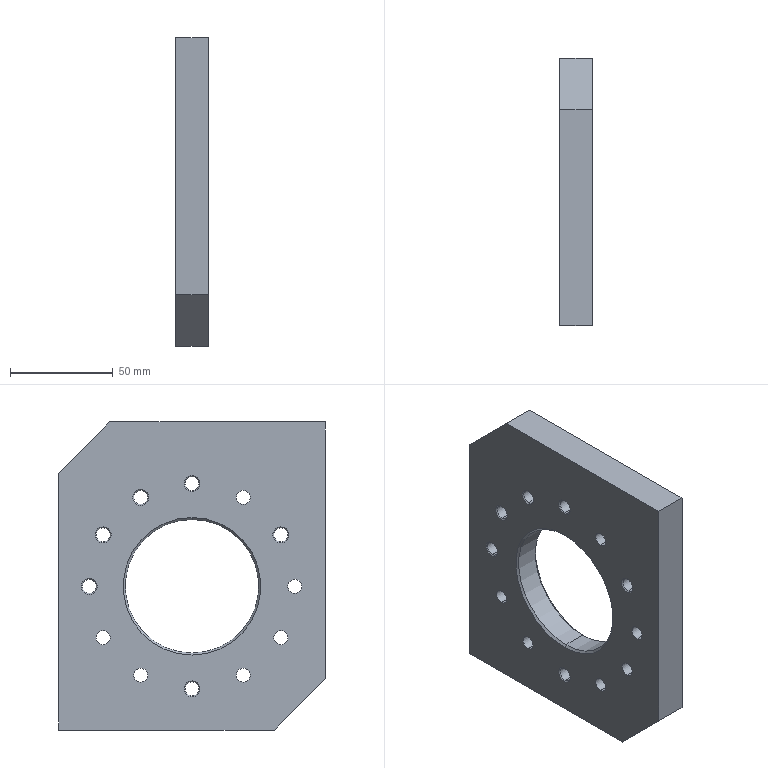Component | SolidWorks | THK-A1023DrivenWheelMountingPlateRight-1 | 1 solid | 65 faces | box 16 x 130 x 150 mm | volume 224529 mm3 | cone 28 | cylinder 28 | plane 9 | commonest cylinder face diameters 6.8 x24 125 x2 65 x2 | material 45
build123d program:
from build123d import *

# Parameters (mm, degrees)
SKETCH1_W           = 150
SKETCH1_H           = 130
BOSS_EXTRUDE1_DEPTH = 8
SKETCH2_R           = 32.5
CUT_EXTRUDE1_DEPTH  = 101.529
SKETCH3_R           = 62.5
CUT_EXTRUDE2_DEPTH  = 2
M8_TAPPED_HOLE1_D   = 6.8
CHAMFER1_SIZE       = 25
CHAMFER2_SIZE       = 1.5
CHAMFER3_SIZE       = 1
CHAMFER4_SIZE       = 0.5
CHAMFER5_SIZE       = 25


with BuildPart() as part:
    # Sketch1 → Boss-Extrude1 (new, symmetric)
    with BuildSketch(Plane(origin=(0, 0, 0), x_dir=(0, 0, -1), z_dir=(1, 0, 0))):
        Rectangle(SKETCH1_W, SKETCH1_H)
    extrude(amount=BOSS_EXTRUDE1_DEPTH, both=True)

    # Sketch2 → Cut-Extrude1 (cut, through all)
    with BuildSketch(Plane.ZY.offset(8)):
        with Locations((-5, 0)):
            Circle(SKETCH2_R)
    extrude(amount=-CUT_EXTRUDE1_DEPTH, mode=Mode.SUBTRACT)

    # Sketch3 → Cut-Extrude2 (cut)
    with BuildSketch(Plane.ZY.offset(-8)):
        with Locations((-5, 0)):
            Circle(SKETCH3_R)
    extrude(amount=CUT_EXTRUDE2_DEPTH, mode=Mode.SUBTRACT)

    # M8 Tapped Hole1 (through all)
    with Locations(Plane(origin=(6, 0, 0), x_dir=(0, 0, -1), z_dir=(1, 0, 0))):
        with Locations((5, 50), (-45, 0), (-20, -43.301), (-20, 43.301), (-38.301, 25), (55, 0), (30, 43.301), (30, -43.301), (5, -50), (48.301, -25), (48.301, 25), (-38.301, -25)):
            Hole(M8_TAPPED_HOLE1_D / 2)

    # Chamfer1
    chamfer1_edges = [part.edges().sort_by_distance(p)[0] for p in [
        (0, -65, -75),
    ]]
    chamfer(chamfer1_edges, length=CHAMFER1_SIZE)

    # Chamfer2
    chamfer2_edges = [part.edges().sort_by_distance(p)[0] for p in [
        (6, 0, -37.5),
    ]]
    chamfer(chamfer2_edges, length=CHAMFER2_SIZE)

    # Chamfer3
    chamfer3_edges = [part.edges().sort_by_distance(p)[0] for p in [
        (-8, 0, -37.5),
    ]]
    chamfer(chamfer3_edges, length=CHAMFER3_SIZE)

    # Chamfer4
    chamfer4_edges = [part.edges().sort_by_distance(p)[0] for p in [
        (6, 0, -58.4),
        (-8, 0, -58.4),
        (6, 25, 34.901),
        (-8, 25, 34.901),
        (6, 43.301, 16.6),
        (-8, 43.301, 16.6),
        (6, -43.301, 16.6),
        (-8, -43.301, 16.6),
        (6, 0, 41.6),
        (-8, 0, 41.6),
        (6, 50, -8.4),
        (-8, 50, -8.4),
    ]]
    chamfer(chamfer4_edges, length=CHAMFER4_SIZE)

    # Chamfer5
    chamfer5_edges = [part.edges().sort_by_distance(p)[0] for p in [
        (0, 65, 75),
    ]]
    chamfer(chamfer5_edges, length=CHAMFER5_SIZE)


solid = part.part

# Placed as in the assembly
solid = solid.moved(Location((65, -95, -1324), (0, 0, 0)))